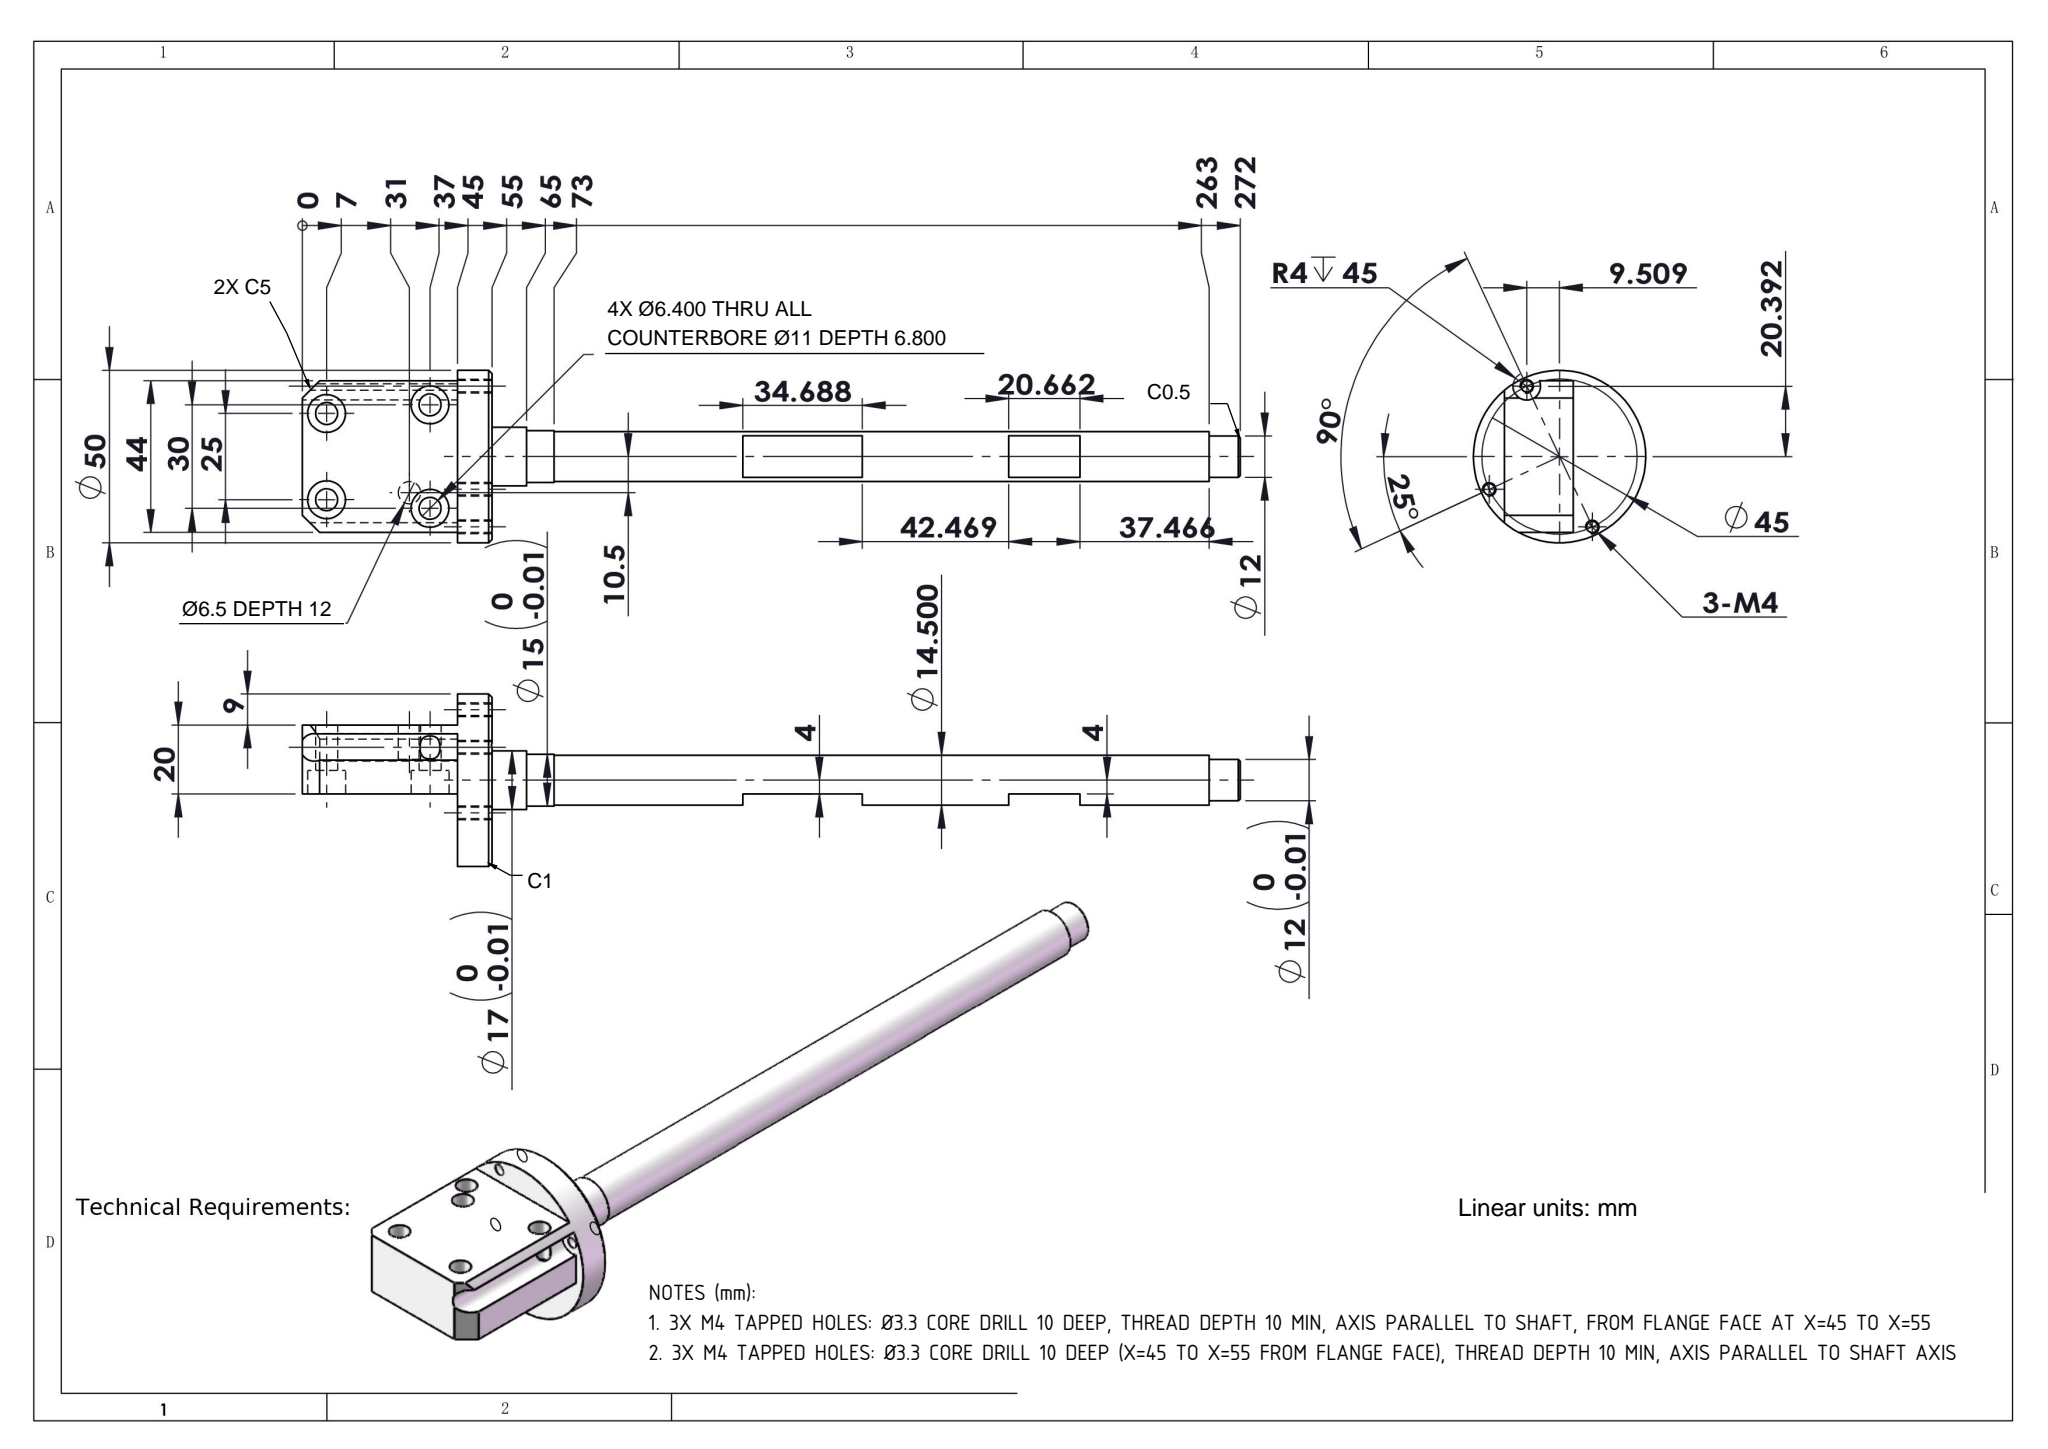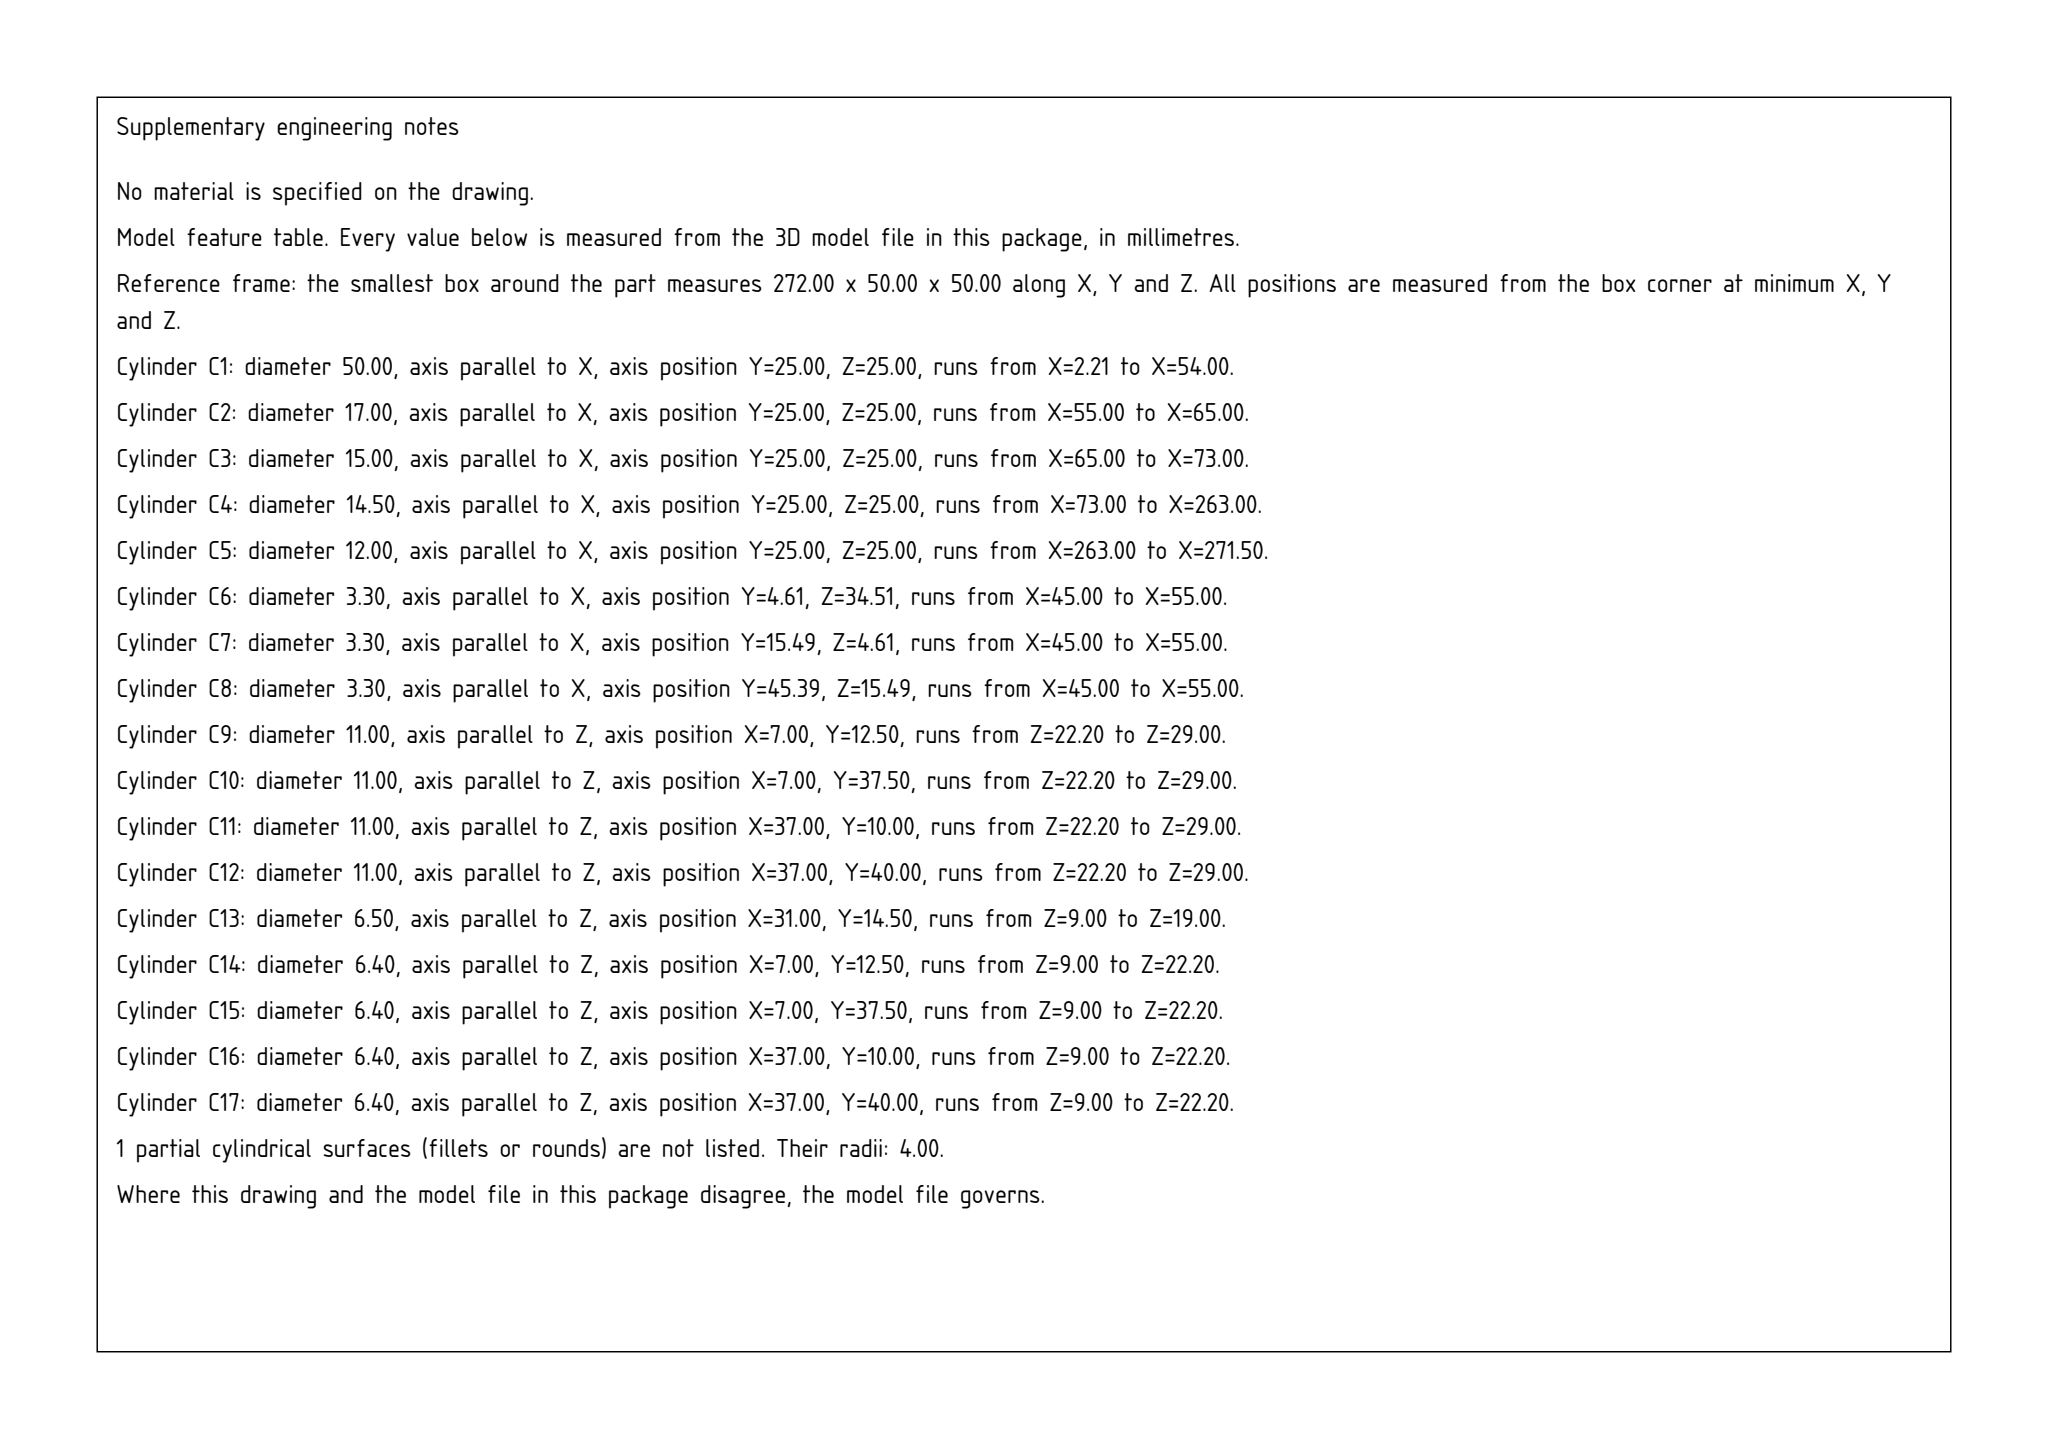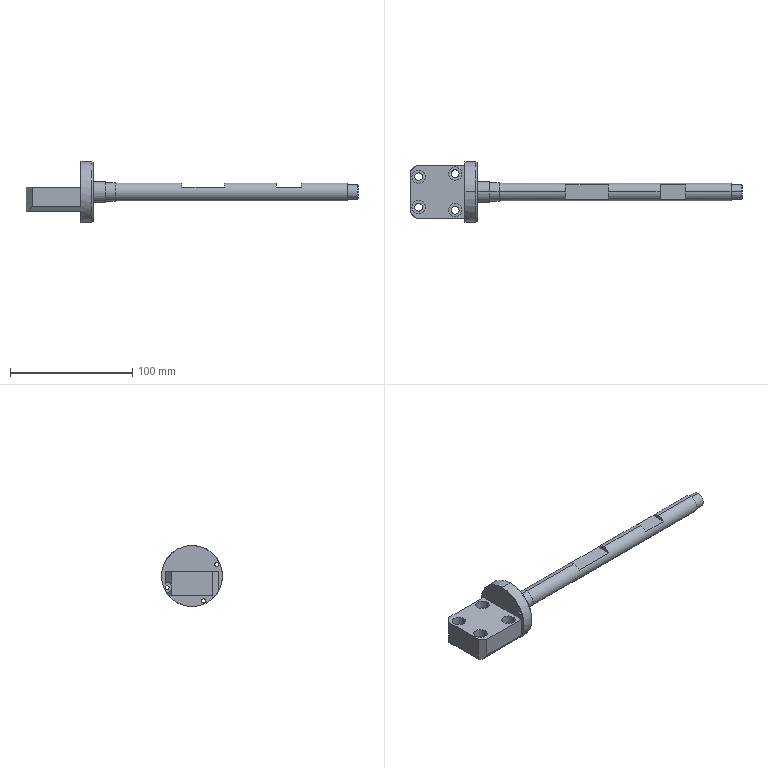Part | SolidWorks | mm | 1 solid | 67 faces | box 272 x 50 x 50 mm | volume 86347 mm3 | cylinder 37 | plane 26 | cone 4 | commonest cylinder face diameters 11 x8 6.4 x8 3.3 x6 8 x3 12 x2 6.5 x2 17 x2 50 x2
Drawing notes:
3X M4 TAPPED HOLES: Ø3.3 CORE DRILL 10 DEEP, THREAD DEPTH 10 MIN, AXIS PARALLEL TO SHAFT, FROM FLANGE FACE AT X=45 TO X=55 | from the solid: cylinders: hole/bore Ø3.3, axis x, from 45.0 to 55.0 (3 instances at y/z = [15.5,4.6], [4.6,34.5], [45.4,15.5])
3X M4 TAPPED HOLES: Ø3.3 CORE DRILL 10 DEEP (X=45 TO X=55 FROM FLANGE FACE), THREAD DEPTH 10 MIN, AXIS PARALLEL TO SHAFT AXIS | from the solid: cylinders: hole/bore Ø3.3, axis x, from 45.0 to 55.0 (3 instances at y/z = 15.5/4.6, 4.6/34.5, 45.4/15.5)